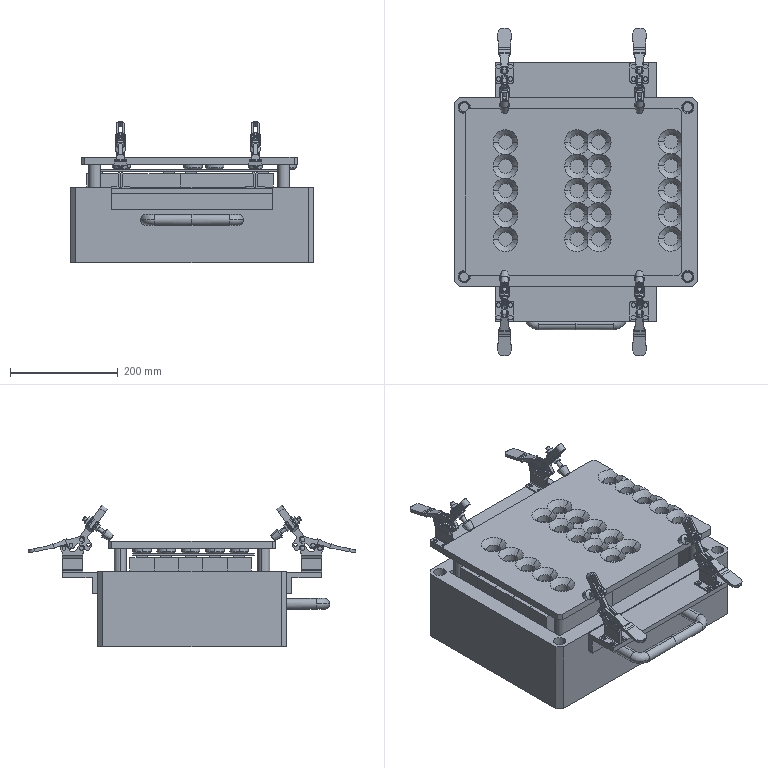Assembly | SolidWorks | mm | 61 component files | 61 solids | 1739 faces | box 450 x 607.53 x 263.06 mm | volume 22996457 mm3 | plane 955 | cylinder 548 | cone 208 | spline 24 | torus 4 | commonest cylinder face diameters 6.35 x64 34 x40 26 x40 8 x40 12.8 x36 7.35 x32 6.7 x32 6 x28
Bill of materials:
AD12-160328-001K.SDPRT | 2 |  | Straight extruded bar with an L-shaped (angle) cross-section and unequal legs: one wide flat flange and one shorter perpendicular leg.
AD12-CompressionSpring.SDPRT | 4 |  | Helical coil spring made of round-section wire, with roughly 9-10 active coils at what looks like a constant pitch and straight cylindrical outer envelope.
AD12-daozhu.SDPRT | 4 |  | Solid plain right circular cylinder (rod or pin blank) with flat ends, several times longer than its diameter.
AD12-Handle.SDPRT | 2 |  | Solid round rod bent through about 90 degrees with a generous bend radius, giving two straight legs that end in flat square-cut faces.
AD12-huiiuban.SDPRT | 1 |  | Thin flat rectangular plate or sheet with no holes or features.
AD12-_MC01H-4_bo.sdprt | 4 |  | Axisymmetric stepped pin: a slender cylindrical shank joined to a larger head shaped as a conical frustum, which tapers away from the shank.
AD12-_MC01H-4_bod.sdprt | 4 |  | Bracket that looks like folded sheet: a rectangular base flange with four obround slots, and a vertical web made of two back-to-back layers. At the top the two layers split into a Y-shaped clevis with two lobed ears, and cylindrical cross pins pass through both ear pairs.
AD12-_MC01H-4_c.sdprt | 4 |  | Thick obround (stadium-shaped) link plate with two round through holes, one near the center of each rounded end.
AD12-_MC01H-4_h.sdprt | 4 |  | Hexagonal prism with a central round through bore, with chamfered corners on the faces (hex-nut-like shape).
AD12-_MC01H-4_n.sdprt | 8 |  | Flat bar link or lever with a long closed slot at one rounded end, a narrower stepped neck, and an angled, bent end tab with two small round holes.
AD12-_MC01H-4_s.sdprt | 4 |  | Curved sheet clip or saddle: a cylindrically curved plate with a central round hole, two straight parallel side legs, and concave curved end edges.
AD12-_MC01H-4_w.sdprt | 8 |  | Lever or handle with a broad flat paddle at one end, a tapering arm, and a forked clevis end made of two parallel plates. Two cylindrical cross pins span the plates. In side profile the arm curves into a lobed end.
AD12-SquareCell.SDPRT | 10 | 6061-T6 (SS) | Thin rectangular box-shaped solid with two small raised rectangular tabs near opposite ends of the narrow top face; each tab carries a shallow surface marking, one a single line (minus-like) and the other a cross (plus-like).
AD12-SquareCellJig.SDPRT | 1 | 6061-T6 (SS) | Rectangular open-top tray or box housing with a deep rectangular pocket, a flat rim around the top, chamfered vertical corners, and one round hole in the rim at each of the four corners.
AD12-SquareCellPressPlate.SDPRT | 1 |  | Thin flat rectangular plate with small corner chamfers and 20 countersunk round holes in four columns of five. Two columns sit close together near the middle, one is near the left edge, and the column at the right edge is cut open by the plate edge.
Mates:
1. coincident | AD12-SquareCell.SDPRT-15 face at (-374.414, -78.961, 324.12) dir (0, 1, 0) | AD12-SquareCell.SDPRT-25 face at (-374.414, -78.961, 324.12) dir (0, -1, 0)
2. coincident | AD12-SquareCell.SDPRT-25 face at (-374.414, -33.961, 324.12) dir (0, 1, 0) | AD12-SquareCell.SDPRT-27 face at (-374.414, -33.961, 324.12) dir (0, -1, 0)
3. coincident | assembly face at (-191.414, -38.961, 319.12) dir (-1, 0, 0) | AD12-SquareCell.SDPRT-27 face at (-201.414, -33.961, 324.12) dir (1, 0, 0)
4. coincident | AD12-SquareCell.SDPRT-27 face at (-374.414, 11.039, 324.12) dir (0, 1, 0) | AD12-SquareCell.SDPRT-29 face at (-374.414, 11.039, 324.12) dir (0, -1, 0)
5. coincident | AD12-SquareCell.SDPRT-27 face at (-374.414, -33.961, 324.12) dir (-1, 0, 0) | AD12-SquareCell.SDPRT-29 face at (-374.414, 11.039, 324.12) dir (-1, 0, 0)
6. coincident | AD12-SquareCell.SDPRT-29 face at (-374.414, 56.039, 324.12) dir (0, 1, 0) | AD12-SquareCell.SDPRT-31 face at (-374.414, 56.039, 324.12) dir (0, -1, 0)
7. coincident | assembly face at (-191.414, -38.961, 199.12) dir (0, 0, -1) | AD12-SquareCellJig.SDPRT-1 face at (-179.414, -13.961, 199.12) dir (0, 0, 1)
8. coincident | AD12-SquareCell.SDPRT-29 face at (-374.414, 11.039, 324.12) dir (0, 0, 1) | AD12-SquareCell.SDPRT-31 face at (-374.414, 56.039, 324.12) dir (0, 0, 1)
9. coincident | AD12-SquareCell.SDPRT-27 face at (-374.414, -33.961, 324.12) dir (0, 0, 1) | AD12-SquareCell.SDPRT-29 face at (-374.414, 11.039, 324.12) dir (0, 0, 1)
10. coincident | AD12-SquareCell.SDPRT-25 face at (-374.414, -78.961, 324.12) dir (0, 0, 1) | AD12-SquareCell.SDPRT-27 face at (-374.414, -33.961, 324.12) dir (0, 0, 1)
11. coincident | AD12-SquareCellJig.SDPRT-1 face at (-374.414, -158.961, 199.12) dir (1, 0, 0) | AD12-SquareCell.SDPRT-15 face at (-374.414, -123.961, 324.12) dir (-1, 0, 0)
12. concentric | AD12-SquareCellJig.SDPRT-1 face at (-386.414, 143.039, 209.12) dir (0, 0, 1) r 11.5 | AD12-CompressionSpring.SDPRT-1 face at (-386.414, 143.039, 205.363) dir (0, 0, 1) r 9.629
13. concentric | AD12-SquareCellJig.SDPRT-1 face at (-386.414, -170.961, 209.12) dir (0, 0, 1) r 11.5 | AD12-CompressionSpring.SDPRT-2 face at (-386.414, -170.961, 205.363) dir (0, 0, 1) r 9.629
14. concentric | AD12-SquareCellJig.SDPRT-1 face at (27.586, -170.961, 209.12) dir (0, 0, 1) r 11.5 | AD12-CompressionSpring.SDPRT-3 face at (27.586, -170.961, 205.363) dir (0, 0, 1) r 9.629
15. coincident | AD12-daozhu.SDPRT-1 face at (-359.414, 119.039, 344.12) dir (0, 0, 1) | AD12-SquareCellPressPlate.SDPRT-1 edge at (-359.414, 119.039, 344.12) dir (0, 0, -1) r 11
16. coincident | AD12-daozhu.SDPRT-4 edge at (-9.414, -146.961, 344.12) dir (0, 0, 1) r 11 | AD12-SquareCellPressPlate.SDPRT-1 edge at (-9.414, -146.961, 344.12) dir (0, 0, -1) r 11
17. coincident | AD12-SquareCellJig.SDPRT-1 face at (-404.414, -188.961, 299.12) dir (0, -1, 0) | AD12-Handle.SDPRT-5 face at (-264.414, -188.961, 239.12) dir (0, 1, 0)
18. concentric | AD12-Handle.SDPRT-5 face at (-249.414, -258.961, 239.12) dir (1, 0, 0) r 10 | AD12-Handle.SDPRT-6 face at (-109.414, -258.961, 239.12) dir (-1, 0, 0) r 10
19. coincident | AD12-Handle.SDPRT-5 edge at (-179.414, -258.961, 239.12) dir (1, 0, 0) r 10 | AD12-Handle.SDPRT-6 edge at (-179.414, -258.961, 239.12) dir (-1, 0, 0) r 10
20. coincident | AD12-SquareCellJig.SDPRT-1 face at (-404.414, -188.961, 299.12) dir (0, -1, 0) | AD12-Handle.SDPRT-5 face at (-264.414, -188.961, 239.12) dir (0, 1, 0)
21. coincident | AD12-Handle.SDPRT-5 face at (-264.414, -188.961, 239.12) dir (0, 1, 0) | AD12-Handle.SDPRT-6 face at (-94.414, -188.961, 239.12) dir (0, 1, 0)
22. distance | AD12-Handle.SDPRT-5 plane at (-179.414, -258.961, 239.12) dir (0, 0, 1) | AD12-SquareCellJig.SDPRT-1 plane at (-179.414, -13.961, 159.12) dir (0, 0, 1)
23. coincident | AD12-SquareCellJig.SDPRT-1 plane at (-179.414, -13.961, 159.12) dir (1, 0, 0) | AD12-Handle.SDPRT-6 plane at (-179.414, -258.961, 239.12) dir (-1, 0, 0)
24. coincident | AD12-huiiuban.SDPRT-1 face at (-191.414, -16.461, 332.12) dir (0, 0, 1) | AD12-SquareCellPressPlate.SDPRT-1 face at (-310.147, 78.531, 332.12) dir (0, 0, -1)
25. coincident | AD12-SquareCell.SDPRT-31 face at (-374.414, 56.039, 329.12) dir (0, 0, 1) | AD12-huiiuban.SDPRT-1 face at (-191.414, -16.461, 329.12) dir (0, 0, -1)
26. coincident | AD12-SquareCellJig.SDPRT-1 face at (-179.414, -13.961, 199.12) dir (0, 0, 1) | AD12-SquareCell.SDPRT-32 face at (-201.414, 56.039, 199.12) dir (0, 0, -1)
27. coincident | AD12-SquareCellJig.SDPRT-1 face at (-404.414, -188.961, 299.12) dir (0, -1, 0) | AD12-160328-001K.SDPRT-1 face at (-329.414, -188.961, 297.437) dir (0, 1, 0)
28. parallel | AD12-SquareCellJig.SDPRT-1 face at (-179.414, -13.961, 299.12) dir (0, 0, 1) | AD12-160328-001K.SDPRT-1 face at (-329.414, -253.961, 297.437) dir (0, 0, 1)
29. coincident | AD12-SquareCellJig.SDPRT-1 plane at (-179.414, -13.961, 159.12) dir (1, 0, 0) | AD12-160328-001K.SDPRT-1 plane at (-179.414, -253.961, 297.437) dir (-1, 0, 0)
30. coincident | AD12-SquareCellJig.SDPRT-1 face at (-404.414, 161.039, 299.12) dir (0, 1, 0) | AD12-160328-001K.SDPRT-2 face at (-29.414, 161.039, 297.437) dir (0, -1, 0)
31. coincident | AD12-160328-001K.SDPRT-1 face at (-329.414, -253.961, 297.437) dir (0, 0, 1) | AD12-160328-001K.SDPRT-2 face at (-29.414, 226.039, 297.437) dir (0, 0, 1)
32. coincident | AD12-SquareCellJig.SDPRT-1 plane at (-179.414, -13.961, 159.12) dir (1, 0, 0) | AD12-160328-001K.SDPRT-2 plane at (-179.414, 226.039, 297.437) dir (1, 0, 0)
33. coincident | AD12-160328-001K.SDPRT-1 face at (-329.414, -253.961, 297.437) dir (0, 0, 1) | AD12-MC01H-4_2_03.SDASM-1/AD12-_MC01H-4_bod.sdprt-1 face at (-294.414, -234.961, 297.437) dir (0, 0, -1)
34. coincident | AD12-160328-001K.SDPRT-1 face at (-329.414, -253.961, 297.437) dir (-1, 0, 0) | AD12-MC01H-4_2_03.SDASM-1/AD12-_MC01H-4_bod.sdprt-1 face at (-329.414, -264.961, 300.437) dir (-1, 0, 0)
35. coincident | AD12-160328-001K.SDPRT-1 face at (-329.414, -253.961, 287.437) dir (0, -1, 0) | AD12-MC01H-4_2_03.SDASM-1/AD12-_MC01H-4_bod.sdprt-1 face at (-345.014, -253.961, 297.437) dir (0, -1, 0)
36. coincident | AD12-SquareCell.SDPRT-26 face at (-28.414, -78.961, 324.12) dir (1, 0, 0) | AD12-SquareCell.SDPRT-24 face at (-28.414, -123.961, 324.12) dir (1, 0, 0)
37. coincident | AD12-SquareCell.SDPRT-30 face at (-28.414, 11.039, 324.12) dir (1, 0, 0) | AD12-SquareCell.SDPRT-24 face at (-28.414, -123.961, 324.12) dir (1, 0, 0)
38. coincident | AD12-SquareCell.SDPRT-32 face at (-28.414, 56.039, 324.12) dir (1, 0, 0) | AD12-SquareCell.SDPRT-28 face at (-28.414, -33.961, 324.12) dir (1, 0, 0)
39. distance | AD12-SquareCellJig.SDPRT-1 face at (-374.414, -158.961, 199.12) dir (0, 1, 0) | AD12-SquareCell.SDPRT-15 face at (-374.414, -123.961, 324.12) dir (0, -1, 0)
40. distance | AD12-_MC01H-4_w.sdprt-2 face at (-29.886, 75.189, 24.85) dir (0.8137, 0.5813, 0) | AD12-_MC01H-4_s.sdprt-1 face at (-49.976, 118.76, 17.5) dir (0.8137, 0.5813, 0)
41. distance | AD12-_MC01H-4_w.sdprt-2 face at (-29.886, 75.189, 26.02) dir (0, 0, 1) | AD12-_MC01H-4_s.sdprt-1 face at (-55.117, 65.745, 24.85) dir (0, 0, 1)
42. coincident | AD12-_MC01H-4_n.sdprt-2 face at (-43.195, 84.116, 17.5) dir (0.8137, 0.5813, 0) | AD12-_MC01H-4_w.sdprt-2 face at (-34.475, 71.911, 27.5) dir (-0.8137, -0.5813, 0)
43. coincident | AD12-_MC01H-4_n.sdprt-1 face at (-29.736, 93.731, 17.5) dir (-0.8137, -0.5813, 0) | AD12-_MC01H-4_w.sdprt-1 face at (-21.017, 81.525, 7.5) dir (0.8137, 0.5813, 0)
44. coincident | AD12-_MC01H-4_s.sdprt-1 face at (-49.976, 118.76, 17.5) dir (0.8137, 0.5813, 0) | AD12-_MC01H-4_w.sdprt-1 face at (-22.579, 80.409, 24.85) dir (-0.8137, -0.5813, 0)
45. distance | AD12-_MC01H-4_w.sdprt-1 face at (-23.946, 79.433, 26.02) dir (0, 0, 1) | AD12-_MC01H-4_s.sdprt-1 face at (-55.117, 65.745, 24.85) dir (0, 0, 1)
46. distance | AD12-_MC01H-4_bo.sdprt-1 face at (-20.411, 100.392, 17.5) dir (0.8137, 0.5813, 0) | AD12-_MC01H-4_n.sdprt-1 face at (-21.903, 91.367, 18.052) dir (0.8137, 0.5813, 0)
47. concentric | AD12-_MC01H-4_s.sdprt-1 face at (-16.15, 60.4, 20.5) dir (0, 0, -1) r 3.175 | AD12-_MC01H-4_h.sdprt-1 face at (-16.15, 60.4, 67.5) dir (0, 0, -1) r 3.175
48. coincident | AD12-_MC01H-4_w.sdprt-1 face at (-32.508, 80.407, 23.557) dir (0.5813, -0.8137, 0) | AD12-_MC01H-4_w.sdprt-2 face at (-29.692, 82.419, 26.02) dir (0.5813, -0.8137, 0)
49. concentric | AD12-_MC01H-4_bo.sdprt-1 face at (-71.674, 63.771, 17.5) dir (0.8137, 0.5813, 0) r 4 | AD12-_MC01H-4_w.sdprt-1 face at (-29.736, 93.731, 17.5) dir (-0.8137, -0.5813, 0) r 4
50. coincident | AD12-_MC01H-4_bod.sdprt-1 face at (30, 31.745, 20.5) dir (0, 0, -1) | AD12-_MC01H-4_s.sdprt-1 face at (-20.483, 17.265, 20.5) dir (0, 0, 1)
51. concentric | AD12-_MC01H-4_bo.sdprt-1 face at (-71.674, 63.771, 17.5) dir (0.8137, 0.5813, 0) r 4 | AD12-_MC01H-4_n.sdprt-1 face at (-35.839, 89.371, 17.5) dir (0.8137, 0.5813, 0) r 4
52. concentric | AD12-_MC01H-4_bo.sdprt-1 face at (-71.674, 63.771, 17.5) dir (0.8137, 0.5813, 0) r 4 | AD12-_MC01H-4_n.sdprt-2 face at (-37.092, 88.476, 17.5) dir (-0.8137, -0.5813, 0) r 4